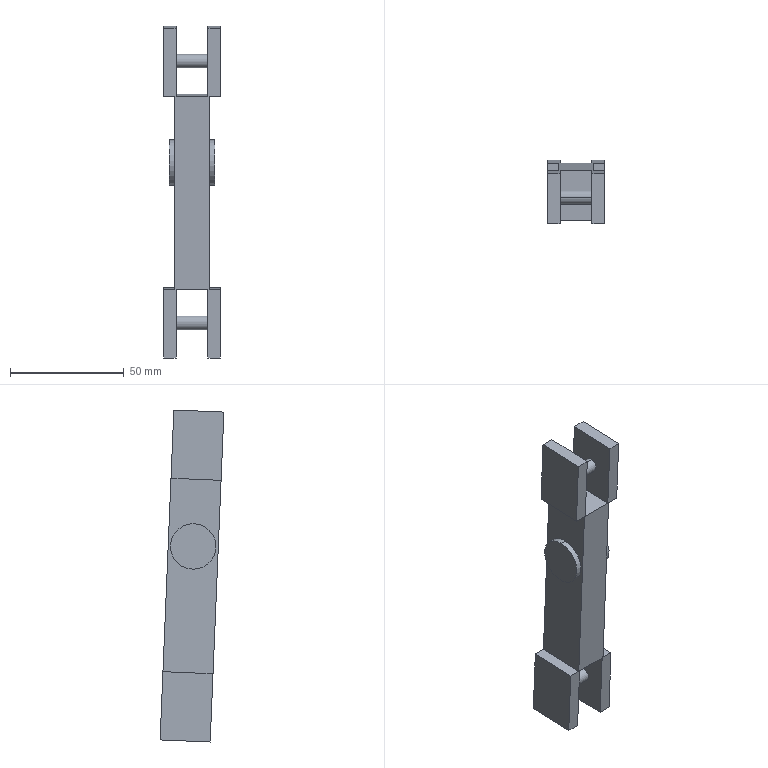Component | SolidWorks | HZ022-A001-D007-1 | 1 solid | 32 faces | box 25 x 28.01 x 145.79 mm | volume 44932 mm3 | plane 24 | cylinder 8 | commonest cylinder face diameters 20 x4 6 x4 | material AL6061
build123d program:
from build123d import *

# Parameters (mm, degrees)
SKETCH1_W           = 22
SKETCH1_H           = 115
BOSS_EXTRUDE1_DEPTH = 7.5
SKETCH3_W           = 22
SKETCH3_H           = 30
BOSS_EXTRUDE2_DEPTH = 12.5
SKETCH4_W           = 22
SKETCH4_H           = 30
SKETCH4_R           = 3
CUT_EXTRUDE1_DEPTH  = 7
SKETCH5_R           = 10
BOSS_EXTRUDE3_DEPTH = 10


with BuildPart() as part:
    # Sketch1 → Boss-Extrude1 (new, symmetric)
    with BuildSketch(Plane(origin=(0, 0, 0), x_dir=(1, 0, 0), z_dir=(0, 1, 0))):
        Rectangle(SKETCH1_W, SKETCH1_H)
    extrude(amount=BOSS_EXTRUDE1_DEPTH, both=True)

    # Sketch3 → Boss-Extrude2 (add, symmetric)
    with BuildSketch(Plane(origin=(0, 0, 0), x_dir=(1, 0, 0), z_dir=(0, 1, 0))):
        with Locations((0, 57.5)):
            Rectangle(SKETCH3_W, SKETCH3_H)
        with Locations((0, -57.5)):
            Rectangle(SKETCH3_W, SKETCH3_H)
    extrude(amount=BOSS_EXTRUDE2_DEPTH, both=True)

    # Sketch4 → Cut-Extrude1 (cut, symmetric)
    # profile 1 of 2: a face of its own
    with BuildSketch(Plane(origin=(0, 0, 0), x_dir=(1, 0, 0), z_dir=(0, 1, 0))):
        with Locations((0, 57.5)):
            Rectangle(SKETCH4_W, SKETCH4_H)
        with Locations(Location((0, 57.5, 0), (0, 0, 270))):
            Circle(SKETCH4_R, mode=Mode.SUBTRACT)
    # profile 2 of 2: a face of its own
    with BuildSketch(Plane(origin=(0, 0, 0), x_dir=(1, 0, 0), z_dir=(0, 1, 0))):
        with Locations((0, -57.5)):
            Rectangle(SKETCH4_W, SKETCH4_H)
        with Locations(Location((0, -57.5, 0), (0, 0, 90))):
            Circle(SKETCH4_R, mode=Mode.SUBTRACT)
    extrude(amount=CUT_EXTRUDE1_DEPTH, both=True, mode=Mode.SUBTRACT)

    # Sketch5 → Boss-Extrude3 (add, symmetric)
    with BuildSketch(Plane(origin=(0, 0, 0), x_dir=(1, 0, 0), z_dir=(0, 1, 0))):
        with Locations(Location((0, -13, 0), (0, 0, 270))):
            Circle(SKETCH5_R)
    extrude(amount=BOSS_EXTRUDE3_DEPTH, both=True)


solid = part.part

# Placed as in the assembly
solid = solid.moved(Location((-12.865, 48.938, 423.011), (2.381, 0, 90)))
STEP:
#1=CARTESIAN_POINT('',(-0.1128,1.889,17.559));
#2=VERTEX_POINT('',#1);
#3=CARTESIAN_POINT('',(-0.1128,1.922,16.772));
#4=VERTEX_POINT('',#3);
#5=CARTESIAN_POINT('',(-0.1128,1.905,17.165));
#6=DIRECTION('',(1.,-0.,-0.));
#7=DIRECTION('',(0.,-0.04155,0.9991));
#8=AXIS2_PLACEMENT_3D('',#5,#6,#7);
#9=CIRCLE('',#8,0.3937);
#10=EDGE_CURVE('',#2,#4,#9,.T.);
#11=ORIENTED_EDGE('',*,*,#10,.F.);
#12=CARTESIAN_POINT('',(-0.2112,1.889,17.559));
#13=VERTEX_POINT('',#12);
#14=CARTESIAN_POINT('',(-0.1128,1.889,17.559));
#15=DIRECTION('',(-1.,0.,0.));
#16=VECTOR('',#15,39.37);
#17=LINE('',#14,#16);
#18=EDGE_CURVE('',#2,#13,#17,.T.);
#19=ORIENTED_EDGE('',*,*,#18,.T.);
#20=CARTESIAN_POINT('',(-0.2112,1.922,16.772));
#21=VERTEX_POINT('',#20);
#22=CARTESIAN_POINT('',(-0.2112,1.905,17.165));
#23=DIRECTION('',(-1.,0.,0.));
#24=DIRECTION('',(0.,-0.04155,0.9991));
#25=AXIS2_PLACEMENT_3D('',#22,#23,#24);
#26=CIRCLE('',#25,0.3937);
#27=EDGE_CURVE('',#21,#13,#26,.T.);
#28=ORIENTED_EDGE('',*,*,#27,.F.);
#29=CARTESIAN_POINT('',(-0.1128,1.922,16.772));
#30=DIRECTION('',(-1.,0.,0.));
#31=VECTOR('',#30,39.37);
#32=LINE('',#29,#31);
#33=EDGE_CURVE('',#4,#21,#32,.T.);
#34=ORIENTED_EDGE('',*,*,#33,.F.);
#35=EDGE_LOOP('',(#11,#19,#28,#34));
#36=FACE_OUTER_BOUND('',#35,.T.);
#37=CARTESIAN_POINT('',(-0.1128,1.905,17.165));
#38=DIRECTION('',(-1.,0.,0.));
#39=DIRECTION('',(0.,0.04155,-0.9991));
#40=AXIS2_PLACEMENT_3D('',#37,#38,#39);
#41=CYLINDRICAL_SURFACE('',#40,0.3937);
#42=ADVANCED_FACE('',(#36),#41,.T.);
#43=CARTESIAN_POINT('',(-0.8018,1.922,16.772));
#44=VERTEX_POINT('',#43);
#45=CARTESIAN_POINT('',(-0.8018,1.889,17.559));
#46=VERTEX_POINT('',#45);
#47=CARTESIAN_POINT('',(-0.8018,1.905,17.165));
#48=DIRECTION('',(-1.,0.,0.));
#49=DIRECTION('',(0.,-0.04155,0.9991));
#50=AXIS2_PLACEMENT_3D('',#47,#48,#49);
#51=CIRCLE('',#50,0.3937);
#52=EDGE_CURVE('',#44,#46,#51,.T.);
#53=ORIENTED_EDGE('',*,*,#52,.T.);
#54=CARTESIAN_POINT('',(-0.9002,1.889,17.559));
#55=VERTEX_POINT('',#54);
#56=CARTESIAN_POINT('',(-0.1128,1.889,17.559));
#57=DIRECTION('',(-1.,0.,0.));
#58=VECTOR('',#57,39.37);
#59=LINE('',#56,#58);
#60=EDGE_CURVE('',#46,#55,#59,.T.);
#61=ORIENTED_EDGE('',*,*,#60,.T.);
#62=CARTESIAN_POINT('',(-0.9002,1.922,16.772));
#63=VERTEX_POINT('',#62);
#64=CARTESIAN_POINT('',(-0.9002,1.905,17.165));
#65=DIRECTION('',(1.,-0.,-0.));
#66=DIRECTION('',(0.,-0.04155,0.9991));
#67=AXIS2_PLACEMENT_3D('',#64,#65,#66);
#68=CIRCLE('',#67,0.3937);
#69=EDGE_CURVE('',#55,#63,#68,.T.);
#70=ORIENTED_EDGE('',*,*,#69,.T.);
#71=CARTESIAN_POINT('',(-0.1128,1.922,16.772));
#72=DIRECTION('',(-1.,0.,0.));
#73=VECTOR('',#72,39.37);
#74=LINE('',#71,#73);
#75=EDGE_CURVE('',#44,#63,#74,.T.);
#76=ORIENTED_EDGE('',*,*,#75,.F.);
#77=EDGE_LOOP('',(#53,#61,#70,#76));
#78=FACE_OUTER_BOUND('',#77,.T.);
#79=CARTESIAN_POINT('',(-0.1128,1.905,17.165));
#80=DIRECTION('',(-1.,0.,0.));
#81=DIRECTION('',(0.,0.04155,-0.9991));
#82=AXIS2_PLACEMENT_3D('',#79,#80,#81);
#83=CYLINDRICAL_SURFACE('',#82,0.3937);
#84=ADVANCED_FACE('',(#78),#83,.T.);
#85=CARTESIAN_POINT('',(-0.7821,2.016,14.51));
#86=VERTEX_POINT('',#85);
#87=CARTESIAN_POINT('',(-0.7821,2.026,14.274));
#88=VERTEX_POINT('',#87);
#89=CARTESIAN_POINT('',(-0.7821,2.021,14.392));
#90=DIRECTION('',(1.,-0.,-0.));
#91=DIRECTION('',(0.,-0.04155,0.9991));
#92=AXIS2_PLACEMENT_3D('',#89,#90,#91);
#93=CIRCLE('',#92,0.1181);
#94=EDGE_CURVE('',#86,#88,#93,.T.);
#95=ORIENTED_EDGE('',*,*,#94,.T.);
#96=CARTESIAN_POINT('',(-0.2309,2.026,14.274));
#97=VERTEX_POINT('',#96);
#98=CARTESIAN_POINT('',(-0.7821,2.026,14.274));
#99=DIRECTION('',(1.,-0.,-0.));
#100=VECTOR('',#99,39.37);
#101=LINE('',#98,#100);
#102=EDGE_CURVE('',#88,#97,#101,.T.);
#103=ORIENTED_EDGE('',*,*,#102,.T.);
#104=CARTESIAN_POINT('',(-0.2309,2.016,14.51));
#105=VERTEX_POINT('',#104);
#106=CARTESIAN_POINT('',(-0.2309,2.021,14.392));
#107=DIRECTION('',(1.,-0.,-0.));
#108=DIRECTION('',(0.,-0.04155,0.9991));
#109=AXIS2_PLACEMENT_3D('',#106,#107,#108);
#110=CIRCLE('',#109,0.1181);
#111=EDGE_CURVE('',#105,#97,#110,.T.);
#112=ORIENTED_EDGE('',*,*,#111,.F.);
#113=CARTESIAN_POINT('',(-0.7821,2.016,14.51));
#114=DIRECTION('',(1.,-0.,-0.));
#115=VECTOR('',#114,39.37);
#116=LINE('',#113,#115);
#117=EDGE_CURVE('',#86,#105,#116,.T.);
#118=ORIENTED_EDGE('',*,*,#117,.F.);
#119=EDGE_LOOP('',(#95,#103,#112,#118));
#120=FACE_OUTER_BOUND('',#119,.T.);
#121=CARTESIAN_POINT('',(-0.7821,2.021,14.392));
#122=DIRECTION('',(1.,-0.,-0.));
#123=DIRECTION('',(0.,-0.04155,0.9991));
#124=AXIS2_PLACEMENT_3D('',#121,#122,#123);
#125=CYLINDRICAL_SURFACE('',#124,0.1181);
#126=ADVANCED_FACE('',(#120),#125,.T.);
#127=CARTESIAN_POINT('',(-0.7821,1.828,19.034));
#128=VERTEX_POINT('',#127);
#129=CARTESIAN_POINT('',(-0.7821,1.838,18.798));
#130=VERTEX_POINT('',#129);
#131=CARTESIAN_POINT('',(-0.7821,1.833,18.916));
#132=DIRECTION('',(1.,-0.,-0.));
#133=DIRECTION('',(0.,0.04155,-0.9991));
#134=AXIS2_PLACEMENT_3D('',#131,#132,#133);
#135=CIRCLE('',#134,0.1181);
#136=EDGE_CURVE('',#128,#130,#135,.T.);
#137=ORIENTED_EDGE('',*,*,#136,.T.);
#138=CARTESIAN_POINT('',(-0.2309,1.838,18.798));
#139=VERTEX_POINT('',#138);
#140=CARTESIAN_POINT('',(-0.7821,1.838,18.798));
#141=DIRECTION('',(1.,-0.,-0.));
#142=VECTOR('',#141,39.37);
#143=LINE('',#140,#142);
#144=EDGE_CURVE('',#130,#139,#143,.T.);
#145=ORIENTED_EDGE('',*,*,#144,.T.);
#146=CARTESIAN_POINT('',(-0.2309,1.828,19.034));
#147=VERTEX_POINT('',#146);
#148=CARTESIAN_POINT('',(-0.2309,1.833,18.916));
#149=DIRECTION('',(1.,-0.,-0.));
#150=DIRECTION('',(0.,0.04155,-0.9991));
#151=AXIS2_PLACEMENT_3D('',#148,#149,#150);
#152=CIRCLE('',#151,0.1181);
#153=EDGE_CURVE('',#147,#139,#152,.T.);
#154=ORIENTED_EDGE('',*,*,#153,.F.);
#155=CARTESIAN_POINT('',(-0.7821,1.828,19.034));
#156=DIRECTION('',(1.,-0.,-0.));
#157=VECTOR('',#156,39.37);
#158=LINE('',#155,#157);
#159=EDGE_CURVE('',#128,#147,#158,.T.);
#160=ORIENTED_EDGE('',*,*,#159,.F.);
#161=EDGE_LOOP('',(#137,#145,#154,#160));
#162=FACE_OUTER_BOUND('',#161,.T.);
#163=CARTESIAN_POINT('',(-0.7821,1.833,18.916));
#164=DIRECTION('',(1.,-0.,-0.));
#165=DIRECTION('',(0.,-0.04155,0.9991));
#166=AXIS2_PLACEMENT_3D('',#163,#164,#165);
#167=CYLINDRICAL_SURFACE('',#166,0.1181);
#168=ADVANCED_FACE('',(#162),#167,.T.);
#169=CARTESIAN_POINT('',(-0.7821,1.564,14.964));
#170=VERTEX_POINT('',#169);
#171=CARTESIAN_POINT('',(-0.7821,1.613,13.784));
#172=VERTEX_POINT('',#171);
#173=CARTESIAN_POINT('',(-0.7821,1.613,13.784));
#174=DIRECTION('',(0.,0.04155,-0.9991));
#175=VECTOR('',#174,39.37);
#176=LINE('',#173,#175);
#177=EDGE_CURVE('',#170,#172,#176,.T.);
#178=ORIENTED_EDGE('',*,*,#177,.F.);
#179=CARTESIAN_POINT('',(-0.2309,1.564,14.964));
#180=VERTEX_POINT('',#179);
#181=CARTESIAN_POINT('',(-0.7821,1.564,14.964));
#182=DIRECTION('',(1.,-0.,-0.));
#183=VECTOR('',#182,39.37);
#184=LINE('',#181,#183);
#185=EDGE_CURVE('',#170,#180,#184,.T.);
#186=ORIENTED_EDGE('',*,*,#185,.T.);
#187=CARTESIAN_POINT('',(-0.2309,1.613,13.784));
#188=VERTEX_POINT('',#187);
#189=CARTESIAN_POINT('',(-0.2309,1.613,13.784));
#190=DIRECTION('',(0.,0.04155,-0.9991));
#191=VECTOR('',#190,39.37);
#192=LINE('',#189,#191);
#193=EDGE_CURVE('',#180,#188,#192,.T.);
#194=ORIENTED_EDGE('',*,*,#193,.T.);
#195=CARTESIAN_POINT('',(-0.01437,1.613,13.784));
#196=VERTEX_POINT('',#195);
#197=CARTESIAN_POINT('',(-0.01437,1.613,13.784));
#198=DIRECTION('',(-1.,0.,0.));
#199=VECTOR('',#198,39.37);
#200=LINE('',#197,#199);
#201=EDGE_CURVE('',#196,#188,#200,.T.);
#202=ORIENTED_EDGE('',*,*,#201,.F.);
#203=CARTESIAN_POINT('',(-0.01437,1.564,14.964));
#204=VERTEX_POINT('',#203);
#205=CARTESIAN_POINT('',(-0.01437,1.613,13.784));
#206=DIRECTION('',(0.,0.04155,-0.9991));
#207=VECTOR('',#206,39.37);
#208=LINE('',#205,#207);
#209=EDGE_CURVE('',#204,#196,#208,.T.);
#210=ORIENTED_EDGE('',*,*,#209,.F.);
#211=CARTESIAN_POINT('',(-0.2112,1.564,14.964));
#212=VERTEX_POINT('',#211);
#213=CARTESIAN_POINT('',(-0.01437,1.564,14.964));
#214=DIRECTION('',(-1.,0.,0.));
#215=VECTOR('',#214,39.37);
#216=LINE('',#213,#215);
#217=EDGE_CURVE('',#204,#212,#216,.T.);
#218=ORIENTED_EDGE('',*,*,#217,.T.);
#219=CARTESIAN_POINT('',(-0.2112,1.424,18.308));
#220=VERTEX_POINT('',#219);
#221=CARTESIAN_POINT('',(-0.2112,1.588,14.374));
#222=DIRECTION('',(0.,0.04155,-0.9991));
#223=VECTOR('',#222,39.37);
#224=LINE('',#221,#223);
#225=EDGE_CURVE('',#220,#212,#224,.T.);
#226=ORIENTED_EDGE('',*,*,#225,.F.);
#227=CARTESIAN_POINT('',(-0.01437,1.424,18.308));
#228=VERTEX_POINT('',#227);
#229=CARTESIAN_POINT('',(-0.01437,1.424,18.308));
#230=DIRECTION('',(-1.,0.,0.));
#231=VECTOR('',#230,39.37);
#232=LINE('',#229,#231);
#233=EDGE_CURVE('',#228,#220,#232,.T.);
#234=ORIENTED_EDGE('',*,*,#233,.F.);
#235=CARTESIAN_POINT('',(-0.01437,1.375,19.488));
#236=VERTEX_POINT('',#235);
#237=CARTESIAN_POINT('',(-0.01437,1.375,19.488));
#238=DIRECTION('',(0.,0.04155,-0.9991));
#239=VECTOR('',#238,39.37);
#240=LINE('',#237,#239);
#241=EDGE_CURVE('',#236,#228,#240,.T.);
#242=ORIENTED_EDGE('',*,*,#241,.F.);
#243=CARTESIAN_POINT('',(-0.2309,1.375,19.488));
#244=VERTEX_POINT('',#243);
#245=CARTESIAN_POINT('',(-0.01437,1.375,19.488));
#246=DIRECTION('',(-1.,0.,0.));
#247=VECTOR('',#246,39.37);
#248=LINE('',#245,#247);
#249=EDGE_CURVE('',#236,#244,#248,.T.);
#250=ORIENTED_EDGE('',*,*,#249,.T.);
#251=CARTESIAN_POINT('',(-0.2309,1.424,18.308));
#252=VERTEX_POINT('',#251);
#253=CARTESIAN_POINT('',(-0.2309,1.375,19.488));
#254=DIRECTION('',(0.,0.04155,-0.9991));
#255=VECTOR('',#254,39.37);
#256=LINE('',#253,#255);
#257=EDGE_CURVE('',#244,#252,#256,.T.);
#258=ORIENTED_EDGE('',*,*,#257,.T.);
#259=CARTESIAN_POINT('',(-0.7821,1.424,18.308));
#260=VERTEX_POINT('',#259);
#261=CARTESIAN_POINT('',(-0.7821,1.424,18.308));
#262=DIRECTION('',(1.,-0.,-0.));
#263=VECTOR('',#262,39.37);
#264=LINE('',#261,#263);
#265=EDGE_CURVE('',#260,#252,#264,.T.);
#266=ORIENTED_EDGE('',*,*,#265,.F.);
#267=CARTESIAN_POINT('',(-0.7821,1.375,19.488));
#268=VERTEX_POINT('',#267);
#269=CARTESIAN_POINT('',(-0.7821,1.375,19.488));
#270=DIRECTION('',(0.,0.04155,-0.9991));
#271=VECTOR('',#270,39.37);
#272=LINE('',#269,#271);
#273=EDGE_CURVE('',#268,#260,#272,.T.);
#274=ORIENTED_EDGE('',*,*,#273,.F.);
#275=CARTESIAN_POINT('',(-0.9986,1.375,19.488));
#276=VERTEX_POINT('',#275);
#277=CARTESIAN_POINT('',(-0.01437,1.375,19.488));
#278=DIRECTION('',(-1.,0.,0.));
#279=VECTOR('',#278,39.37);
#280=LINE('',#277,#279);
#281=EDGE_CURVE('',#268,#276,#280,.T.);
#282=ORIENTED_EDGE('',*,*,#281,.T.);
#283=CARTESIAN_POINT('',(-0.9986,1.424,18.308));
#284=VERTEX_POINT('',#283);
#285=CARTESIAN_POINT('',(-0.9986,1.375,19.488));
#286=DIRECTION('',(0.,0.04155,-0.9991));
#287=VECTOR('',#286,39.37);
#288=LINE('',#285,#287);
#289=EDGE_CURVE('',#276,#284,#288,.T.);
#290=ORIENTED_EDGE('',*,*,#289,.T.);
#291=CARTESIAN_POINT('',(-0.8018,1.424,18.308));
#292=VERTEX_POINT('',#291);
#293=CARTESIAN_POINT('',(-0.01437,1.424,18.308));
#294=DIRECTION('',(-1.,0.,0.));
#295=VECTOR('',#294,39.37);
#296=LINE('',#293,#295);
#297=EDGE_CURVE('',#292,#284,#296,.T.);
#298=ORIENTED_EDGE('',*,*,#297,.F.);
#299=CARTESIAN_POINT('',(-0.8018,1.564,14.964));
#300=VERTEX_POINT('',#299);
#301=CARTESIAN_POINT('',(-0.8018,1.588,14.374));
#302=DIRECTION('',(0.,0.04155,-0.9991));
#303=VECTOR('',#302,39.37);
#304=LINE('',#301,#303);
#305=EDGE_CURVE('',#292,#300,#304,.T.);
#306=ORIENTED_EDGE('',*,*,#305,.T.);
#307=CARTESIAN_POINT('',(-0.9986,1.564,14.964));
#308=VERTEX_POINT('',#307);
#309=CARTESIAN_POINT('',(-0.01437,1.564,14.964));
#310=DIRECTION('',(-1.,0.,0.));
#311=VECTOR('',#310,39.37);
#312=LINE('',#309,#311);
#313=EDGE_CURVE('',#300,#308,#312,.T.);
#314=ORIENTED_EDGE('',*,*,#313,.T.);
#315=CARTESIAN_POINT('',(-0.9986,1.613,13.784));
#316=VERTEX_POINT('',#315);
#317=CARTESIAN_POINT('',(-0.9986,1.613,13.784));
#318=DIRECTION('',(0.,0.04155,-0.9991));
#319=VECTOR('',#318,39.37);
#320=LINE('',#317,#319);
#321=EDGE_CURVE('',#308,#316,#320,.T.);
#322=ORIENTED_EDGE('',*,*,#321,.T.);
#323=CARTESIAN_POINT('',(-0.01437,1.613,13.784));
#324=DIRECTION('',(-1.,0.,0.));
#325=VECTOR('',#324,39.37);
#326=LINE('',#323,#325);
#327=EDGE_CURVE('',#172,#316,#326,.T.);
#328=ORIENTED_EDGE('',*,*,#327,.F.);
#329=EDGE_LOOP('',(#178,#186,#194,#202,#210,#218,#226,#234,#242,#250,#258,#266,#274,#282,#290,#298,#306,#314,#322,#328));
#330=FACE_OUTER_BOUND('',#329,.T.);
#331=CARTESIAN_POINT('',(-0.2112,1.588,14.374));
#332=DIRECTION('',(0.,0.9991,0.04155));
#333=DIRECTION('',(-0.,-0.04155,0.9991));
#334=AXIS2_PLACEMENT_3D('',#331,#332,#333);
#335=PLANE('',#334);
#336=ADVANCED_FACE('',(#330),#335,.F.);
#337=CARTESIAN_POINT('',(-0.7821,2.478,13.82));
#338=VERTEX_POINT('',#337);
#339=CARTESIAN_POINT('',(-0.7821,2.429,15.));
#340=VERTEX_POINT('',#339);
#341=CARTESIAN_POINT('',(-0.7821,2.478,13.82));
#342=DIRECTION('',(-0.,-0.04155,0.9991));
#343=VECTOR('',#342,39.37);
#344=LINE('',#341,#343);
#345=EDGE_CURVE('',#338,#340,#344,.T.);
#346=ORIENTED_EDGE('',*,*,#345,.F.);
#347=CARTESIAN_POINT('',(-0.9986,2.478,13.82));
#348=VERTEX_POINT('',#347);
#349=CARTESIAN_POINT('',(-0.01437,2.478,13.82));
#350=DIRECTION('',(-1.,0.,0.));
#351=VECTOR('',#350,39.37);
#352=LINE('',#349,#351);
#353=EDGE_CURVE('',#338,#348,#352,.T.);
#354=ORIENTED_EDGE('',*,*,#353,.T.);
#355=CARTESIAN_POINT('',(-0.9986,2.429,15.));
#356=VERTEX_POINT('',#355);
#357=CARTESIAN_POINT('',(-0.9986,2.478,13.82));
#358=DIRECTION('',(-0.,-0.04155,0.9991));
#359=VECTOR('',#358,39.37);
#360=LINE('',#357,#359);
#361=EDGE_CURVE('',#348,#356,#360,.T.);
#362=ORIENTED_EDGE('',*,*,#361,.T.);
#363=CARTESIAN_POINT('',(-0.8018,2.429,15.));
#364=VERTEX_POINT('',#363);
#365=CARTESIAN_POINT('',(-0.01437,2.429,15.));
#366=DIRECTION('',(-1.,0.,0.));
#367=VECTOR('',#366,39.37);
#368=LINE('',#365,#367);
#369=EDGE_CURVE('',#364,#356,#368,.T.);
#370=ORIENTED_EDGE('',*,*,#369,.F.);
#371=CARTESIAN_POINT('',(-0.8018,2.29,18.344));
#372=VERTEX_POINT('',#371);
#373=CARTESIAN_POINT('',(-0.8018,2.453,14.41));
#374=DIRECTION('',(-0.,-0.04155,0.9991));
#375=VECTOR('',#374,39.37);
#376=LINE('',#373,#375);
#377=EDGE_CURVE('',#364,#372,#376,.T.);
#378=ORIENTED_EDGE('',*,*,#377,.T.);
#379=CARTESIAN_POINT('',(-0.9986,2.29,18.344));
#380=VERTEX_POINT('',#379);
#381=CARTESIAN_POINT('',(-0.01437,2.29,18.344));
#382=DIRECTION('',(-1.,0.,0.));
#383=VECTOR('',#382,39.37);
#384=LINE('',#381,#383);
#385=EDGE_CURVE('',#372,#380,#384,.T.);
#386=ORIENTED_EDGE('',*,*,#385,.T.);
#387=CARTESIAN_POINT('',(-0.9986,2.241,19.524));
#388=VERTEX_POINT('',#387);
#389=CARTESIAN_POINT('',(-0.9986,2.241,19.524));
#390=DIRECTION('',(-0.,-0.04155,0.9991));
#391=VECTOR('',#390,39.37);
#392=LINE('',#389,#391);
#393=EDGE_CURVE('',#380,#388,#392,.T.);
#394=ORIENTED_EDGE('',*,*,#393,.T.);
#395=CARTESIAN_POINT('',(-0.7821,2.241,19.524));
#396=VERTEX_POINT('',#395);
#397=CARTESIAN_POINT('',(-0.01437,2.241,19.524));
#398=DIRECTION('',(-1.,0.,0.));
#399=VECTOR('',#398,39.37);
#400=LINE('',#397,#399);
#401=EDGE_CURVE('',#396,#388,#400,.T.);
#402=ORIENTED_EDGE('',*,*,#401,.F.);
#403=CARTESIAN_POINT('',(-0.7821,2.29,18.344));
#404=VERTEX_POINT('',#403);
#405=CARTESIAN_POINT('',(-0.7821,2.241,19.524));
#406=DIRECTION('',(-0.,-0.04155,0.9991));
#407=VECTOR('',#406,39.37);
#408=LINE('',#405,#407);
#409=EDGE_CURVE('',#404,#396,#408,.T.);
#410=ORIENTED_EDGE('',*,*,#409,.F.);
#411=CARTESIAN_POINT('',(-0.2309,2.29,18.344));
#412=VERTEX_POINT('',#411);
#413=CARTESIAN_POINT('',(-0.7821,2.29,18.344));
#414=DIRECTION('',(1.,-0.,-0.));
#415=VECTOR('',#414,39.37);
#416=LINE('',#413,#415);
#417=EDGE_CURVE('',#404,#412,#416,.T.);
#418=ORIENTED_EDGE('',*,*,#417,.T.);
#419=CARTESIAN_POINT('',(-0.2309,2.241,19.524));
#420=VERTEX_POINT('',#419);
#421=CARTESIAN_POINT('',(-0.2309,2.241,19.524));
#422=DIRECTION('',(-0.,-0.04155,0.9991));
#423=VECTOR('',#422,39.37);
#424=LINE('',#421,#423);
#425=EDGE_CURVE('',#412,#420,#424,.T.);
#426=ORIENTED_EDGE('',*,*,#425,.T.);
#427=CARTESIAN_POINT('',(-0.01437,2.241,19.524));
#428=VERTEX_POINT('',#427);
#429=CARTESIAN_POINT('',(-0.01437,2.241,19.524));
#430=DIRECTION('',(-1.,0.,0.));
#431=VECTOR('',#430,39.37);
#432=LINE('',#429,#431);
#433=EDGE_CURVE('',#428,#420,#432,.T.);
#434=ORIENTED_EDGE('',*,*,#433,.F.);
#435=CARTESIAN_POINT('',(-0.01437,2.29,18.344));
#436=VERTEX_POINT('',#435);
#437=CARTESIAN_POINT('',(-0.01437,2.241,19.524));
#438=DIRECTION('',(-0.,-0.04155,0.9991));
#439=VECTOR('',#438,39.37);
#440=LINE('',#437,#439);
#441=EDGE_CURVE('',#436,#428,#440,.T.);
#442=ORIENTED_EDGE('',*,*,#441,.F.);
#443=CARTESIAN_POINT('',(-0.2112,2.29,18.344));
#444=VERTEX_POINT('',#443);
#445=CARTESIAN_POINT('',(-0.01437,2.29,18.344));
#446=DIRECTION('',(-1.,0.,0.));
#447=VECTOR('',#446,39.37);
#448=LINE('',#445,#447);
#449=EDGE_CURVE('',#436,#444,#448,.T.);
#450=ORIENTED_EDGE('',*,*,#449,.T.);
#451=CARTESIAN_POINT('',(-0.2112,2.429,15.));
#452=VERTEX_POINT('',#451);
#453=CARTESIAN_POINT('',(-0.2112,2.453,14.41));
#454=DIRECTION('',(-0.,-0.04155,0.9991));
#455=VECTOR('',#454,39.37);
#456=LINE('',#453,#455);
#457=EDGE_CURVE('',#452,#444,#456,.T.);
#458=ORIENTED_EDGE('',*,*,#457,.F.);
#459=CARTESIAN_POINT('',(-0.01437,2.429,15.));
#460=VERTEX_POINT('',#459);
#461=CARTESIAN_POINT('',(-0.01437,2.429,15.));
#462=DIRECTION('',(-1.,0.,0.));
#463=VECTOR('',#462,39.37);
#464=LINE('',#461,#463);
#465=EDGE_CURVE('',#460,#452,#464,.T.);
#466=ORIENTED_EDGE('',*,*,#465,.F.);
#467=CARTESIAN_POINT('',(-0.01437,2.478,13.82));
#468=VERTEX_POINT('',#467);
#469=CARTESIAN_POINT('',(-0.01437,2.478,13.82));
#470=DIRECTION('',(-0.,-0.04155,0.9991));
#471=VECTOR('',#470,39.37);
#472=LINE('',#469,#471);
#473=EDGE_CURVE('',#468,#460,#472,.T.);
#474=ORIENTED_EDGE('',*,*,#473,.F.);
#475=CARTESIAN_POINT('',(-0.2309,2.478,13.82));
#476=VERTEX_POINT('',#475);
#477=CARTESIAN_POINT('',(-0.01437,2.478,13.82));
#478=DIRECTION('',(-1.,0.,0.));
#479=VECTOR('',#478,39.37);
#480=LINE('',#477,#479);
#481=EDGE_CURVE('',#468,#476,#480,.T.);
#482=ORIENTED_EDGE('',*,*,#481,.T.);
#483=CARTESIAN_POINT('',(-0.2309,2.429,15.));
#484=VERTEX_POINT('',#483);
#485=CARTESIAN_POINT('',(-0.2309,2.478,13.82));
#486=DIRECTION('',(-0.,-0.04155,0.9991));
#487=VECTOR('',#486,39.37);
#488=LINE('',#485,#487);
#489=EDGE_CURVE('',#476,#484,#488,.T.);
#490=ORIENTED_EDGE('',*,*,#489,.T.);
#491=CARTESIAN_POINT('',(-0.7821,2.429,15.));
#492=DIRECTION('',(1.,-0.,-0.));
#493=VECTOR('',#492,39.37);
#494=LINE('',#491,#493);
#495=EDGE_CURVE('',#340,#484,#494,.T.);
#496=ORIENTED_EDGE('',*,*,#495,.F.);
#497=EDGE_LOOP('',(#346,#354,#362,#370,#378,#386,#394,#402,#410,#418,#426,#434,#442,#450,#458,#466,#474,#482,#490,#496));
#498=FACE_OUTER_BOUND('',#497,.T.);
#499=CARTESIAN_POINT('',(-0.2112,2.453,14.41));
#500=DIRECTION('',(-0.,-0.9991,-0.04155));
#501=DIRECTION('',(0.,0.04155,-0.9991));
#502=AXIS2_PLACEMENT_3D('',#499,#500,#501);
#503=PLANE('',#502);
#504=ADVANCED_FACE('',(#498),#503,.F.);
#505=CARTESIAN_POINT('',(-0.7821,2.478,13.82));
#506=DIRECTION('',(0.,0.9991,0.04155));
#507=VECTOR('',#506,39.37);
#508=LINE('',#505,#507);
#509=EDGE_CURVE('',#172,#338,#508,.T.);
#510=ORIENTED_EDGE('',*,*,#509,.F.);
#511=ORIENTED_EDGE('',*,*,#327,.T.);
#512=CARTESIAN_POINT('',(-0.9986,1.613,13.784));
#513=DIRECTION('',(0.,0.9991,0.04155));
#514=VECTOR('',#513,39.37);
#515=LINE('',#512,#514);
#516=EDGE_CURVE('',#316,#348,#515,.T.);
#517=ORIENTED_EDGE('',*,*,#516,.T.);
#518=ORIENTED_EDGE('',*,*,#353,.F.);
#519=EDGE_LOOP('',(#510,#511,#517,#518));
#520=FACE_OUTER_BOUND('',#519,.T.);
#521=CARTESIAN_POINT('',(-0.01437,1.613,13.784));
#522=DIRECTION('',(-0.,-0.04155,0.9991));
#523=DIRECTION('',(-0.,-0.9991,-0.04155));
#524=AXIS2_PLACEMENT_3D('',#521,#522,#523);
#525=PLANE('',#524);
#526=ADVANCED_FACE('',(#520),#525,.F.);
#527=CARTESIAN_POINT('',(-0.2309,2.241,19.524));
#528=DIRECTION('',(-0.,-0.9991,-0.04155));
#529=VECTOR('',#528,39.37);
#530=LINE('',#527,#529);
#531=EDGE_CURVE('',#420,#244,#530,.T.);
#532=ORIENTED_EDGE('',*,*,#531,.T.);
#533=ORIENTED_EDGE('',*,*,#249,.F.);
#534=CARTESIAN_POINT('',(-0.01437,1.375,19.488));
#535=DIRECTION('',(-0.,-0.9991,-0.04155));
#536=VECTOR('',#535,39.37);
#537=LINE('',#534,#536);
#538=EDGE_CURVE('',#428,#236,#537,.T.);
#539=ORIENTED_EDGE('',*,*,#538,.F.);
#540=ORIENTED_EDGE('',*,*,#433,.T.);
#541=EDGE_LOOP('',(#532,#533,#539,#540));
#542=FACE_OUTER_BOUND('',#541,.T.);
#543=CARTESIAN_POINT('',(-0.01437,1.375,19.488));
#544=DIRECTION('',(0.,0.04155,-0.9991));
#545=DIRECTION('',(0.,0.9991,0.04155));
#546=AXIS2_PLACEMENT_3D('',#543,#544,#545);
#547=PLANE('',#546);
#548=ADVANCED_FACE('',(#542),#547,.F.);
#549=ORIENTED_EDGE('',*,*,#27,.T.);
#550=CARTESIAN_POINT('',(-0.2112,1.905,17.165));
#551=DIRECTION('',(-1.,0.,0.));
#552=DIRECTION('',(0.,-0.04155,0.9991));
#553=AXIS2_PLACEMENT_3D('',#550,#551,#552);
#554=CIRCLE('',#553,0.3937);
#555=EDGE_CURVE('',#13,#21,#554,.T.);
#556=ORIENTED_EDGE('',*,*,#555,.T.);
#557=EDGE_LOOP('',(#549,#556));
#558=FACE_BOUND('',#557,.T.);
#559=ORIENTED_EDGE('',*,*,#457,.T.);
#560=CARTESIAN_POINT('',(-0.2112,1.857,18.326));
#561=DIRECTION('',(-0.,-0.9991,-0.04155));
#562=VECTOR('',#561,39.37);
#563=LINE('',#560,#562);
#564=EDGE_CURVE('',#444,#220,#563,.T.);
#565=ORIENTED_EDGE('',*,*,#564,.T.);
#566=ORIENTED_EDGE('',*,*,#225,.T.);
#567=CARTESIAN_POINT('',(-0.2112,1.996,14.982));
#568=DIRECTION('',(0.,0.9991,0.04155));
#569=VECTOR('',#568,39.37);
#570=LINE('',#567,#569);
#571=EDGE_CURVE('',#212,#452,#570,.T.);
#572=ORIENTED_EDGE('',*,*,#571,.T.);
#573=EDGE_LOOP('',(#559,#565,#566,#572));
#574=FACE_OUTER_BOUND('',#573,.T.);
#575=CARTESIAN_POINT('',(-0.2112,1.927,16.654));
#576=DIRECTION('',(1.,-0.,-0.));
#577=DIRECTION('',(-0.,-0.04155,0.9991));
#578=AXIS2_PLACEMENT_3D('',#575,#576,#577);
#579=PLANE('',#578);
#580=ADVANCED_FACE('',(#558,#574),#579,.T.);
#581=ORIENTED_EDGE('',*,*,#52,.F.);
#582=CARTESIAN_POINT('',(-0.8018,1.905,17.165));
#583=DIRECTION('',(-1.,0.,0.));
#584=DIRECTION('',(0.,-0.04155,0.9991));
#585=AXIS2_PLACEMENT_3D('',#582,#583,#584);
#586=CIRCLE('',#585,0.3937);
#587=EDGE_CURVE('',#46,#44,#586,.T.);
#588=ORIENTED_EDGE('',*,*,#587,.F.);
#589=EDGE_LOOP('',(#581,#588));
#590=FACE_BOUND('',#589,.T.);
#591=CARTESIAN_POINT('',(-0.8018,1.857,18.326));
#592=DIRECTION('',(-0.,-0.9991,-0.04155));
#593=VECTOR('',#592,39.37);
#594=LINE('',#591,#593);
#595=EDGE_CURVE('',#372,#292,#594,.T.);
#596=ORIENTED_EDGE('',*,*,#595,.F.);
#597=ORIENTED_EDGE('',*,*,#377,.F.);
#598=CARTESIAN_POINT('',(-0.8018,1.996,14.982));
#599=DIRECTION('',(0.,0.9991,0.04155));
#600=VECTOR('',#599,39.37);
#601=LINE('',#598,#600);
#602=EDGE_CURVE('',#300,#364,#601,.T.);
#603=ORIENTED_EDGE('',*,*,#602,.F.);
#604=ORIENTED_EDGE('',*,*,#305,.F.);
#605=EDGE_LOOP('',(#596,#597,#603,#604));
#606=FACE_OUTER_BOUND('',#605,.T.);
#607=CARTESIAN_POINT('',(-0.8018,1.927,16.654));
#608=DIRECTION('',(1.,-0.,-0.));
#609=DIRECTION('',(-0.,-0.04155,0.9991));
#610=AXIS2_PLACEMENT_3D('',#607,#608,#609);
#611=PLANE('',#610);
#612=ADVANCED_FACE('',(#590,#606),#611,.F.);
#613=ORIENTED_EDGE('',*,*,#313,.F.);
#614=ORIENTED_EDGE('',*,*,#602,.T.);
#615=ORIENTED_EDGE('',*,*,#369,.T.);
#616=CARTESIAN_POINT('',(-0.9986,1.564,14.964));
#617=DIRECTION('',(-0.,-0.9991,-0.04155));
#618=VECTOR('',#617,39.37);
#619=LINE('',#616,#618);
#620=EDGE_CURVE('',#356,#308,#619,.T.);
#621=ORIENTED_EDGE('',*,*,#620,.T.);
#622=EDGE_LOOP('',(#613,#614,#615,#621));
#623=FACE_OUTER_BOUND('',#622,.T.);
#624=CARTESIAN_POINT('',(-0.01437,1.564,14.964));
#625=DIRECTION('',(0.,0.04155,-0.9991));
#626=DIRECTION('',(0.,0.9991,0.04155));
#627=AXIS2_PLACEMENT_3D('',#624,#625,#626);
#628=PLANE('',#627);
#629=ADVANCED_FACE('',(#623),#628,.F.);
#630=ORIENTED_EDGE('',*,*,#571,.F.);
#631=ORIENTED_EDGE('',*,*,#217,.F.);
#632=CARTESIAN_POINT('',(-0.01437,1.564,14.964));
#633=DIRECTION('',(-0.,-0.9991,-0.04155));
#634=VECTOR('',#633,39.37);
#635=LINE('',#632,#634);
#636=EDGE_CURVE('',#460,#204,#635,.T.);
#637=ORIENTED_EDGE('',*,*,#636,.F.);
#638=ORIENTED_EDGE('',*,*,#465,.T.);
#639=EDGE_LOOP('',(#630,#631,#637,#638));
#640=FACE_OUTER_BOUND('',#639,.T.);
#641=CARTESIAN_POINT('',(-0.01437,1.564,14.964));
#642=DIRECTION('',(0.,0.04155,-0.9991));
#643=DIRECTION('',(0.,0.9991,0.04155));
#644=AXIS2_PLACEMENT_3D('',#641,#642,#643);
#645=PLANE('',#644);
#646=ADVANCED_FACE('',(#640),#645,.F.);
#647=ORIENTED_EDGE('',*,*,#201,.T.);
#648=CARTESIAN_POINT('',(-0.2309,2.478,13.82));
#649=DIRECTION('',(0.,0.9991,0.04155));
#650=VECTOR('',#649,39.37);
#651=LINE('',#648,#650);
#652=EDGE_CURVE('',#188,#476,#651,.T.);
#653=ORIENTED_EDGE('',*,*,#652,.T.);
#654=ORIENTED_EDGE('',*,*,#481,.F.);
#655=CARTESIAN_POINT('',(-0.01437,1.613,13.784));
#656=DIRECTION('',(0.,0.9991,0.04155));
#657=VECTOR('',#656,39.37);
#658=LINE('',#655,#657);
#659=EDGE_CURVE('',#196,#468,#658,.T.);
#660=ORIENTED_EDGE('',*,*,#659,.F.);
#661=EDGE_LOOP('',(#647,#653,#654,#660));
#662=FACE_OUTER_BOUND('',#661,.T.);
#663=CARTESIAN_POINT('',(-0.01437,1.613,13.784));
#664=DIRECTION('',(-0.,-0.04155,0.9991));
#665=DIRECTION('',(-0.,-0.9991,-0.04155));
#666=AXIS2_PLACEMENT_3D('',#663,#664,#665);
#667=PLANE('',#666);
#668=ADVANCED_FACE('',(#662),#667,.F.);
#669=ORIENTED_EDGE('',*,*,#473,.T.);
#670=ORIENTED_EDGE('',*,*,#636,.T.);
#671=ORIENTED_EDGE('',*,*,#209,.T.);
#672=ORIENTED_EDGE('',*,*,#659,.T.);
#673=EDGE_LOOP('',(#669,#670,#671,#672));
#674=FACE_OUTER_BOUND('',#673,.T.);
#675=CARTESIAN_POINT('',(-0.01437,1.927,16.654));
#676=DIRECTION('',(-1.,0.,0.));
#677=DIRECTION('',(0.,0.04155,-0.9991));
#678=AXIS2_PLACEMENT_3D('',#675,#676,#677);
#679=PLANE('',#678);
#680=ADVANCED_FACE('',(#674),#679,.F.);
#681=ORIENTED_EDGE('',*,*,#361,.F.);
#682=ORIENTED_EDGE('',*,*,#516,.F.);
#683=ORIENTED_EDGE('',*,*,#321,.F.);
#684=ORIENTED_EDGE('',*,*,#620,.F.);
#685=EDGE_LOOP('',(#681,#682,#683,#684));
#686=FACE_OUTER_BOUND('',#685,.T.);
#687=CARTESIAN_POINT('',(-0.9986,1.927,16.654));
#688=DIRECTION('',(-1.,0.,0.));
#689=DIRECTION('',(0.,0.04155,-0.9991));
#690=AXIS2_PLACEMENT_3D('',#687,#688,#689);
#691=PLANE('',#690);
#692=ADVANCED_FACE('',(#686),#691,.T.);
#693=ORIENTED_EDGE('',*,*,#385,.F.);
#694=ORIENTED_EDGE('',*,*,#595,.T.);
#695=ORIENTED_EDGE('',*,*,#297,.T.);
#696=CARTESIAN_POINT('',(-0.9986,1.424,18.308));
#697=DIRECTION('',(0.,0.9991,0.04155));
#698=VECTOR('',#697,39.37);
#699=LINE('',#696,#698);
#700=EDGE_CURVE('',#284,#380,#699,.T.);
#701=ORIENTED_EDGE('',*,*,#700,.T.);
#702=EDGE_LOOP('',(#693,#694,#695,#701));
#703=FACE_OUTER_BOUND('',#702,.T.);
#704=CARTESIAN_POINT('',(-0.01437,1.424,18.308));
#705=DIRECTION('',(-0.,-0.04155,0.9991));
#706=DIRECTION('',(-0.,-0.9991,-0.04155));
#707=AXIS2_PLACEMENT_3D('',#704,#705,#706);
#708=PLANE('',#707);
#709=ADVANCED_FACE('',(#703),#708,.F.);
#710=ORIENTED_EDGE('',*,*,#564,.F.);
#711=ORIENTED_EDGE('',*,*,#449,.F.);
#712=CARTESIAN_POINT('',(-0.01437,1.424,18.308));
#713=DIRECTION('',(0.,0.9991,0.04155));
#714=VECTOR('',#713,39.37);
#715=LINE('',#712,#714);
#716=EDGE_CURVE('',#228,#436,#715,.T.);
#717=ORIENTED_EDGE('',*,*,#716,.F.);
#718=ORIENTED_EDGE('',*,*,#233,.T.);
#719=EDGE_LOOP('',(#710,#711,#717,#718));
#720=FACE_OUTER_BOUND('',#719,.T.);
#721=CARTESIAN_POINT('',(-0.01437,1.424,18.308));
#722=DIRECTION('',(-0.,-0.04155,0.9991));
#723=DIRECTION('',(-0.,-0.9991,-0.04155));
#724=AXIS2_PLACEMENT_3D('',#721,#722,#723);
#725=PLANE('',#724);
#726=ADVANCED_FACE('',(#720),#725,.F.);
#727=ORIENTED_EDGE('',*,*,#281,.F.);
#728=CARTESIAN_POINT('',(-0.7821,2.241,19.524));
#729=DIRECTION('',(-0.,-0.9991,-0.04155));
#730=VECTOR('',#729,39.37);
#731=LINE('',#728,#730);
#732=EDGE_CURVE('',#396,#268,#731,.T.);
#733=ORIENTED_EDGE('',*,*,#732,.F.);
#734=ORIENTED_EDGE('',*,*,#401,.T.);
#735=CARTESIAN_POINT('',(-0.9986,1.375,19.488));
#736=DIRECTION('',(-0.,-0.9991,-0.04155));
#737=VECTOR('',#736,39.37);
#738=LINE('',#735,#737);
#739=EDGE_CURVE('',#388,#276,#738,.T.);
#740=ORIENTED_EDGE('',*,*,#739,.T.);
#741=EDGE_LOOP('',(#727,#733,#734,#740));
#742=FACE_OUTER_BOUND('',#741,.T.);
#743=CARTESIAN_POINT('',(-0.01437,1.375,19.488));
#744=DIRECTION('',(0.,0.04155,-0.9991));
#745=DIRECTION('',(0.,0.9991,0.04155));
#746=AXIS2_PLACEMENT_3D('',#743,#744,#745);
#747=PLANE('',#746);
#748=ADVANCED_FACE('',(#742),#747,.F.);
#749=ORIENTED_EDGE('',*,*,#241,.T.);
#750=ORIENTED_EDGE('',*,*,#716,.T.);
#751=ORIENTED_EDGE('',*,*,#441,.T.);
#752=ORIENTED_EDGE('',*,*,#538,.T.);
#753=EDGE_LOOP('',(#749,#750,#751,#752));
#754=FACE_OUTER_BOUND('',#753,.T.);
#755=CARTESIAN_POINT('',(-0.01437,1.927,16.654));
#756=DIRECTION('',(1.,-0.,-0.));
#757=DIRECTION('',(-0.,-0.04155,0.9991));
#758=AXIS2_PLACEMENT_3D('',#755,#756,#757);
#759=PLANE('',#758);
#760=ADVANCED_FACE('',(#754),#759,.T.);
#761=ORIENTED_EDGE('',*,*,#289,.F.);
#762=ORIENTED_EDGE('',*,*,#739,.F.);
#763=ORIENTED_EDGE('',*,*,#393,.F.);
#764=ORIENTED_EDGE('',*,*,#700,.F.);
#765=EDGE_LOOP('',(#761,#762,#763,#764));
#766=FACE_OUTER_BOUND('',#765,.T.);
#767=CARTESIAN_POINT('',(-0.9986,1.927,16.654));
#768=DIRECTION('',(1.,-0.,-0.));
#769=DIRECTION('',(-0.,-0.04155,0.9991));
#770=AXIS2_PLACEMENT_3D('',#767,#768,#769);
#771=PLANE('',#770);
#772=ADVANCED_FACE('',(#766),#771,.F.);
#773=CARTESIAN_POINT('',(-0.2309,2.29,18.344));
#774=DIRECTION('',(0.,0.9991,0.04155));
#775=VECTOR('',#774,39.37);
#776=LINE('',#773,#775);
#777=EDGE_CURVE('',#252,#412,#776,.T.);
#778=ORIENTED_EDGE('',*,*,#777,.T.);
#779=ORIENTED_EDGE('',*,*,#417,.F.);
#780=CARTESIAN_POINT('',(-0.7821,2.29,18.344));
#781=DIRECTION('',(0.,0.9991,0.04155));
#782=VECTOR('',#781,39.37);
#783=LINE('',#780,#782);
#784=EDGE_CURVE('',#260,#404,#783,.T.);
#785=ORIENTED_EDGE('',*,*,#784,.F.);
#786=ORIENTED_EDGE('',*,*,#265,.T.);
#787=EDGE_LOOP('',(#778,#779,#785,#786));
#788=FACE_OUTER_BOUND('',#787,.T.);
#789=CARTESIAN_POINT('',(-0.7821,2.29,18.344));
#790=DIRECTION('',(0.,0.04155,-0.9991));
#791=DIRECTION('',(0.,0.9991,0.04155));
#792=AXIS2_PLACEMENT_3D('',#789,#790,#791);
#793=PLANE('',#792);
#794=ADVANCED_FACE('',(#788),#793,.F.);
#795=ORIENTED_EDGE('',*,*,#136,.F.);
#796=CARTESIAN_POINT('',(-0.7821,1.833,18.916));
#797=DIRECTION('',(1.,-0.,-0.));
#798=DIRECTION('',(0.,0.04155,-0.9991));
#799=AXIS2_PLACEMENT_3D('',#796,#797,#798);
#800=CIRCLE('',#799,0.1181);
#801=EDGE_CURVE('',#130,#128,#800,.T.);
#802=ORIENTED_EDGE('',*,*,#801,.F.);
#803=EDGE_LOOP('',(#795,#802));
#804=FACE_BOUND('',#803,.T.);
#805=ORIENTED_EDGE('',*,*,#409,.T.);
#806=ORIENTED_EDGE('',*,*,#732,.T.);
#807=ORIENTED_EDGE('',*,*,#273,.T.);
#808=ORIENTED_EDGE('',*,*,#784,.T.);
#809=EDGE_LOOP('',(#805,#806,#807,#808));
#810=FACE_OUTER_BOUND('',#809,.T.);
#811=CARTESIAN_POINT('',(-0.7821,1.927,16.654));
#812=DIRECTION('',(-1.,0.,0.));
#813=DIRECTION('',(0.,0.04155,-0.9991));
#814=AXIS2_PLACEMENT_3D('',#811,#812,#813);
#815=PLANE('',#814);
#816=ADVANCED_FACE('',(#804,#810),#815,.F.);
#817=ORIENTED_EDGE('',*,*,#153,.T.);
#818=CARTESIAN_POINT('',(-0.2309,1.833,18.916));
#819=DIRECTION('',(1.,-0.,-0.));
#820=DIRECTION('',(0.,0.04155,-0.9991));
#821=AXIS2_PLACEMENT_3D('',#818,#819,#820);
#822=CIRCLE('',#821,0.1181);
#823=EDGE_CURVE('',#139,#147,#822,.T.);
#824=ORIENTED_EDGE('',*,*,#823,.T.);
#825=EDGE_LOOP('',(#817,#824));
#826=FACE_BOUND('',#825,.T.);
#827=ORIENTED_EDGE('',*,*,#425,.F.);
#828=ORIENTED_EDGE('',*,*,#777,.F.);
#829=ORIENTED_EDGE('',*,*,#257,.F.);
#830=ORIENTED_EDGE('',*,*,#531,.F.);
#831=EDGE_LOOP('',(#827,#828,#829,#830));
#832=FACE_OUTER_BOUND('',#831,.T.);
#833=CARTESIAN_POINT('',(-0.2309,1.927,16.654));
#834=DIRECTION('',(-1.,0.,0.));
#835=DIRECTION('',(0.,0.04155,-0.9991));
#836=AXIS2_PLACEMENT_3D('',#833,#834,#835);
#837=PLANE('',#836);
#838=ADVANCED_FACE('',(#826,#832),#837,.T.);
#839=ORIENTED_EDGE('',*,*,#144,.F.);
#840=ORIENTED_EDGE('',*,*,#801,.T.);
#841=ORIENTED_EDGE('',*,*,#159,.T.);
#842=ORIENTED_EDGE('',*,*,#823,.F.);
#843=EDGE_LOOP('',(#839,#840,#841,#842));
#844=FACE_OUTER_BOUND('',#843,.T.);
#845=CARTESIAN_POINT('',(-0.7821,1.833,18.916));
#846=DIRECTION('',(1.,-0.,-0.));
#847=DIRECTION('',(0.,-0.04155,0.9991));
#848=AXIS2_PLACEMENT_3D('',#845,#846,#847);
#849=CYLINDRICAL_SURFACE('',#848,0.1181);
#850=ADVANCED_FACE('',(#844),#849,.T.);
#851=CARTESIAN_POINT('',(-0.2309,2.429,15.));
#852=DIRECTION('',(-0.,-0.9991,-0.04155));
#853=VECTOR('',#852,39.37);
#854=LINE('',#851,#853);
#855=EDGE_CURVE('',#484,#180,#854,.T.);
#856=ORIENTED_EDGE('',*,*,#855,.T.);
#857=ORIENTED_EDGE('',*,*,#185,.F.);
#858=CARTESIAN_POINT('',(-0.7821,2.429,15.));
#859=DIRECTION('',(-0.,-0.9991,-0.04155));
#860=VECTOR('',#859,39.37);
#861=LINE('',#858,#860);
#862=EDGE_CURVE('',#340,#170,#861,.T.);
#863=ORIENTED_EDGE('',*,*,#862,.F.);
#864=ORIENTED_EDGE('',*,*,#495,.T.);
#865=EDGE_LOOP('',(#856,#857,#863,#864));
#866=FACE_OUTER_BOUND('',#865,.T.);
#867=CARTESIAN_POINT('',(-0.7821,2.429,15.));
#868=DIRECTION('',(-0.,-0.04155,0.9991));
#869=DIRECTION('',(-0.,-0.9991,-0.04155));
#870=AXIS2_PLACEMENT_3D('',#867,#868,#869);
#871=PLANE('',#870);
#872=ADVANCED_FACE('',(#866),#871,.F.);
#873=ORIENTED_EDGE('',*,*,#94,.F.);
#874=CARTESIAN_POINT('',(-0.7821,2.021,14.392));
#875=DIRECTION('',(1.,-0.,-0.));
#876=DIRECTION('',(0.,-0.04155,0.9991));
#877=AXIS2_PLACEMENT_3D('',#874,#875,#876);
#878=CIRCLE('',#877,0.1181);
#879=EDGE_CURVE('',#88,#86,#878,.T.);
#880=ORIENTED_EDGE('',*,*,#879,.F.);
#881=EDGE_LOOP('',(#873,#880));
#882=FACE_BOUND('',#881,.T.);
#883=ORIENTED_EDGE('',*,*,#345,.T.);
#884=ORIENTED_EDGE('',*,*,#862,.T.);
#885=ORIENTED_EDGE('',*,*,#177,.T.);
#886=ORIENTED_EDGE('',*,*,#509,.T.);
#887=EDGE_LOOP('',(#883,#884,#885,#886));
#888=FACE_OUTER_BOUND('',#887,.T.);
#889=CARTESIAN_POINT('',(-0.7821,1.927,16.654));
#890=DIRECTION('',(1.,-0.,-0.));
#891=DIRECTION('',(-0.,-0.04155,0.9991));
#892=AXIS2_PLACEMENT_3D('',#889,#890,#891);
#893=PLANE('',#892);
#894=ADVANCED_FACE('',(#882,#888),#893,.T.);
#895=ORIENTED_EDGE('',*,*,#111,.T.);
#896=CARTESIAN_POINT('',(-0.2309,2.021,14.392));
#897=DIRECTION('',(1.,-0.,-0.));
#898=DIRECTION('',(0.,-0.04155,0.9991));
#899=AXIS2_PLACEMENT_3D('',#896,#897,#898);
#900=CIRCLE('',#899,0.1181);
#901=EDGE_CURVE('',#97,#105,#900,.T.);
#902=ORIENTED_EDGE('',*,*,#901,.T.);
#903=EDGE_LOOP('',(#895,#902));
#904=FACE_BOUND('',#903,.T.);
#905=ORIENTED_EDGE('',*,*,#489,.F.);
#906=ORIENTED_EDGE('',*,*,#652,.F.);
#907=ORIENTED_EDGE('',*,*,#193,.F.);
#908=ORIENTED_EDGE('',*,*,#855,.F.);
#909=EDGE_LOOP('',(#905,#906,#907,#908));
#910=FACE_OUTER_BOUND('',#909,.T.);
#911=CARTESIAN_POINT('',(-0.2309,1.927,16.654));
#912=DIRECTION('',(1.,-0.,-0.));
#913=DIRECTION('',(-0.,-0.04155,0.9991));
#914=AXIS2_PLACEMENT_3D('',#911,#912,#913);
#915=PLANE('',#914);
#916=ADVANCED_FACE('',(#904,#910),#915,.F.);
#917=ORIENTED_EDGE('',*,*,#102,.F.);
#918=ORIENTED_EDGE('',*,*,#879,.T.);
#919=ORIENTED_EDGE('',*,*,#117,.T.);
#920=ORIENTED_EDGE('',*,*,#901,.F.);
#921=EDGE_LOOP('',(#917,#918,#919,#920));
#922=FACE_OUTER_BOUND('',#921,.T.);
#923=CARTESIAN_POINT('',(-0.7821,2.021,14.392));
#924=DIRECTION('',(1.,-0.,-0.));
#925=DIRECTION('',(0.,-0.04155,0.9991));
#926=AXIS2_PLACEMENT_3D('',#923,#924,#925);
#927=CYLINDRICAL_SURFACE('',#926,0.1181);
#928=ADVANCED_FACE('',(#922),#927,.T.);
#929=CARTESIAN_POINT('',(-0.9002,1.905,17.165));
#930=DIRECTION('',(1.,-0.,-0.));
#931=DIRECTION('',(0.,-0.04155,0.9991));
#932=AXIS2_PLACEMENT_3D('',#929,#930,#931);
#933=CIRCLE('',#932,0.3937);
#934=EDGE_CURVE('',#63,#55,#933,.T.);
#935=ORIENTED_EDGE('',*,*,#934,.F.);
#936=ORIENTED_EDGE('',*,*,#69,.F.);
#937=EDGE_LOOP('',(#935,#936));
#938=FACE_OUTER_BOUND('',#937,.T.);
#939=CARTESIAN_POINT('',(-0.9002,1.905,17.165));
#940=DIRECTION('',(1.,-0.,-0.));
#941=DIRECTION('',(-0.,-0.04155,0.9991));
#942=AXIS2_PLACEMENT_3D('',#939,#940,#941);
#943=PLANE('',#942);
#944=ADVANCED_FACE('',(#938),#943,.F.);
#945=ORIENTED_EDGE('',*,*,#60,.F.);
#946=ORIENTED_EDGE('',*,*,#587,.T.);
#947=ORIENTED_EDGE('',*,*,#75,.T.);
#948=ORIENTED_EDGE('',*,*,#934,.T.);
#949=EDGE_LOOP('',(#945,#946,#947,#948));
#950=FACE_OUTER_BOUND('',#949,.T.);
#951=CARTESIAN_POINT('',(-0.1128,1.905,17.165));
#952=DIRECTION('',(-1.,0.,0.));
#953=DIRECTION('',(0.,0.04155,-0.9991));
#954=AXIS2_PLACEMENT_3D('',#951,#952,#953);
#955=CYLINDRICAL_SURFACE('',#954,0.3937);
#956=ADVANCED_FACE('',(#950),#955,.T.);
#957=ORIENTED_EDGE('',*,*,#18,.F.);
#958=CARTESIAN_POINT('',(-0.1128,1.905,17.165));
#959=DIRECTION('',(1.,-0.,-0.));
#960=DIRECTION('',(0.,-0.04155,0.9991));
#961=AXIS2_PLACEMENT_3D('',#958,#959,#960);
#962=CIRCLE('',#961,0.3937);
#963=EDGE_CURVE('',#4,#2,#962,.T.);
#964=ORIENTED_EDGE('',*,*,#963,.F.);
#965=ORIENTED_EDGE('',*,*,#33,.T.);
#966=ORIENTED_EDGE('',*,*,#555,.F.);
#967=EDGE_LOOP('',(#957,#964,#965,#966));
#968=FACE_OUTER_BOUND('',#967,.T.);
#969=CARTESIAN_POINT('',(-0.1128,1.905,17.165));
#970=DIRECTION('',(-1.,0.,0.));
#971=DIRECTION('',(0.,0.04155,-0.9991));
#972=AXIS2_PLACEMENT_3D('',#969,#970,#971);
#973=CYLINDRICAL_SURFACE('',#972,0.3937);
#974=ADVANCED_FACE('',(#968),#973,.T.);
#975=ORIENTED_EDGE('',*,*,#963,.T.);
#976=ORIENTED_EDGE('',*,*,#10,.T.);
#977=EDGE_LOOP('',(#975,#976));
#978=FACE_OUTER_BOUND('',#977,.T.);
#979=CARTESIAN_POINT('',(-0.1128,1.905,17.165));
#980=DIRECTION('',(1.,-0.,-0.));
#981=DIRECTION('',(-0.,-0.04155,0.9991));
#982=AXIS2_PLACEMENT_3D('',#979,#980,#981);
#983=PLANE('',#982);
#984=ADVANCED_FACE('',(#978),#983,.T.);
#985=CLOSED_SHELL('',(#42,#84,#126,#168,#336,#504,#526,#548,#580,#612,#629,#646,#668,#680,#692,#709,#726,#748,#760,#772,#794,#816,#838,#850,#872,#894,#916,#928,#944,#956,#974,#984));
#986=MANIFOLD_SOLID_BREP('',#985);
#987=CARTESIAN_POINT('',(0.,0.,0.));
#988=DIRECTION('',(0.,0.,1.));
#989=DIRECTION('',(1.,0.,0.));
#990=AXIS2_PLACEMENT_3D('',#987,#988,#989);
#991=(LENGTH_UNIT()NAMED_UNIT(*)SI_UNIT($,.METRE.));
#992=LENGTH_MEASURE_WITH_UNIT(LENGTH_MEASURE(0.0254),#991);
#993=DIMENSIONAL_EXPONENTS(1.,0.,0.,0.,0.,0.,0.);
#994=(CONVERSION_BASED_UNIT('',#992)LENGTH_UNIT()NAMED_UNIT(#993));
#995=UNCERTAINTY_MEASURE_WITH_UNIT(LENGTH_MEASURE(0.00001),#994,'','');
#996=(NAMED_UNIT(*)PLANE_ANGLE_UNIT()SI_UNIT($,.RADIAN.));
#997=(NAMED_UNIT(*)SI_UNIT($,.STERADIAN.)SOLID_ANGLE_UNIT());
#998=(GEOMETRIC_REPRESENTATION_CONTEXT(3)GLOBAL_UNCERTAINTY_ASSIGNED_CONTEXT((#995))GLOBAL_UNIT_ASSIGNED_CONTEXT((#994,#996,#997))REPRESENTATION_CONTEXT('',''));
#999=ADVANCED_BREP_SHAPE_REPRESENTATION('',(#986,#990),#998);
#1000=COLOUR_RGB('',0.7922,0.8196,0.9333);
#1001=FILL_AREA_STYLE_COLOUR('',#1000);
#1002=FILL_AREA_STYLE('',(#1001));
#1003=SURFACE_STYLE_FILL_AREA(#1002);
#1004=SURFACE_SIDE_STYLE('',(#1003));
#1005=SURFACE_STYLE_USAGE(.BOTH.,#1004);
#1006=PRESENTATION_STYLE_ASSIGNMENT((#1005));
#1007=STYLED_ITEM('',(#1006),#986);
#1008=PRESENTATION_LAYER_ASSIGNMENT('','',(#1007));
#1009=(LENGTH_UNIT()NAMED_UNIT(*)SI_UNIT($,.METRE.));
#1010=LENGTH_MEASURE_WITH_UNIT(LENGTH_MEASURE(0.0254),#1009);
#1011=DIMENSIONAL_EXPONENTS(1.,0.,0.,0.,0.,0.,0.);
#1012=(CONVERSION_BASED_UNIT('',#1010)LENGTH_UNIT()NAMED_UNIT(#1011));
#1013=UNCERTAINTY_MEASURE_WITH_UNIT(LENGTH_MEASURE(0.00001),#1012,'','');
#1014=(NAMED_UNIT(*)PLANE_ANGLE_UNIT()SI_UNIT($,.RADIAN.));
#1015=(NAMED_UNIT(*)SI_UNIT($,.STERADIAN.)SOLID_ANGLE_UNIT());
#1016=(GEOMETRIC_REPRESENTATION_CONTEXT(3)GLOBAL_UNCERTAINTY_ASSIGNED_CONTEXT((#1013))GLOBAL_UNIT_ASSIGNED_CONTEXT((#1012,#1014,#1015))REPRESENTATION_CONTEXT('',''));
#1017=MECHANICAL_DESIGN_GEOMETRIC_PRESENTATION_REPRESENTATION('',(#1007),#1016);